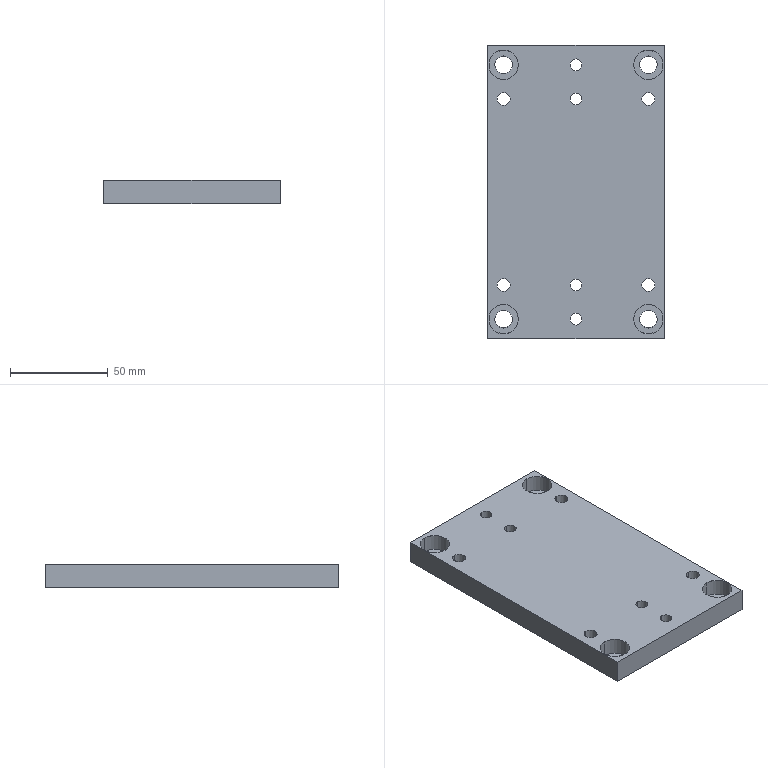Component | SolidWorks | X-AxisSliderShimPlate-1 | 1 solid | 102 faces | box 90 x 150 x 12 mm | volume 150499 mm3 | cone 48 | cylinder 40 | plane 14 | commonest cylinder face diameters 15 x8 9 x8 6 x8 11 x8 6.6 x8
build123d program:
from build123d import *

# Parameters (mm, degrees)
SKETCH1_W                                      = 150
SKETCH1_H                                      = 90
BOSS_EXTRUDE1_DEPTH                            = 12
SKETCH2_R                                      = 3
CUT_EXTRUDE1_DEPTH                             = 89.284
M6_HEX_SOCKET_HEAD_CAP_SCREW_CBORE1_AT_2_COUNT = 2
M6_HEX_SOCKET_HEAD_CAP_SCREW_CBORE1_AT_2_PITCH = 74
M6_HEX_SOCKET_HEAD_CAP_SCREW_CBORE1_AT_3_COUNT = 2
M6_HEX_SOCKET_HEAD_CAP_SCREW_CBORE1_AT_3_PITCH = 120.42
M6_HEX_SOCKET_HEAD_CAP_SCREW_CBORE1_AT_4_COUNT = 2
M6_HEX_SOCKET_HEAD_CAP_SCREW_CBORE1_AT_4_PITCH = 95
SKETCH5_R                                      = 3
CUT_EXTRUDE2_DEPTH                             = 89.284
M8_HEX_SOCKET_HEAD_CAP_SCREW_CBORE1_AT_2_COUNT = 2
M8_HEX_SOCKET_HEAD_CAP_SCREW_CBORE1_AT_2_PITCH = 130
M8_HEX_SOCKET_HEAD_CAP_SCREW_CBORE1_AT_3_COUNT = 2
M8_HEX_SOCKET_HEAD_CAP_SCREW_CBORE1_AT_3_PITCH = 149.586
M8_HEX_SOCKET_HEAD_CAP_SCREW_CBORE1_AT_4_COUNT = 2
M8_HEX_SOCKET_HEAD_CAP_SCREW_CBORE1_AT_4_PITCH = 74


with BuildPart() as part:
    # Sketch1 → Boss-Extrude1 (new body)
    with BuildSketch(Plane.XY):
        Rectangle(SKETCH1_W, SKETCH1_H)
    extrude(amount=BOSS_EXTRUDE1_DEPTH)

    # Sketch2 → Cut-Extrude1 (cut, through all)
    with BuildSketch(Plane.XY.offset(12)):
        with Locations((-47.5, 0)):
            Circle(SKETCH2_R)
        with Locations((47.5, 0)):
            Circle(SKETCH2_R)
    extrude(amount=-CUT_EXTRUDE1_DEPTH, mode=Mode.SUBTRACT)

    # Sketch3 → M6 Hex Socket Head Cap Screw CBORE1 (revolve, cut)
    with BuildSketch(Plane(origin=(-47.5, 37, 12), x_dir=(0, -1, 0), z_dir=(1, 0, 0))):
        Polygon((0, 0), (0, 12), (3.325, 12), (3.3, 11.975), (3.3, 6.425), (3.325, 6.4), (5.5, 6.4), (5.5, 0.025), (5.525, 0), align=None)
    m6_hex_socket_head_cap_screw_cbore1 = revolve(axis=Axis((-47.5, 37, 18.35), (0, 0, -1)), mode=Mode.SUBTRACT)

    # M6 Hex Socket Head Cap Screw CBORE1 at 2: M6 Hex Socket Head Cap Screw CBORE1 ×2
    with Locations(*[(0, -i * M6_HEX_SOCKET_HEAD_CAP_SCREW_CBORE1_AT_2_PITCH, 0) for i in range(1, M6_HEX_SOCKET_HEAD_CAP_SCREW_CBORE1_AT_2_COUNT)]):
        add(m6_hex_socket_head_cap_screw_cbore1, mode=Mode.SUBTRACT)

    # M6 Hex Socket Head Cap Screw CBORE1 at 3: M6 Hex Socket Head Cap Screw CBORE1 ×2
    with Locations(*[Vector(0.7889, -0.6145, 0) * (i * M6_HEX_SOCKET_HEAD_CAP_SCREW_CBORE1_AT_3_PITCH) for i in range(1, M6_HEX_SOCKET_HEAD_CAP_SCREW_CBORE1_AT_3_COUNT)]):
        add(m6_hex_socket_head_cap_screw_cbore1, mode=Mode.SUBTRACT)

    # M6 Hex Socket Head Cap Screw CBORE1 at 4: M6 Hex Socket Head Cap Screw CBORE1 ×2
    with Locations(*[(i * M6_HEX_SOCKET_HEAD_CAP_SCREW_CBORE1_AT_4_PITCH, 0, 0) for i in range(1, M6_HEX_SOCKET_HEAD_CAP_SCREW_CBORE1_AT_4_COUNT)]):
        add(m6_hex_socket_head_cap_screw_cbore1, mode=Mode.SUBTRACT)

    # Sketch5 → Cut-Extrude2 (cut, through all)
    with BuildSketch(Plane(origin=(0, 0, 0), x_dir=(-1, 0, 0), z_dir=(0, 0, -1))):
        with Locations((-65, 0)):
            Circle(SKETCH5_R)
        with Locations((65, 0)):
            Circle(SKETCH5_R)
    extrude(amount=-CUT_EXTRUDE2_DEPTH, mode=Mode.SUBTRACT)

    # Sketch6 → M8 Hex Socket Head Cap Screw CBORE1 (revolve, cut)
    with BuildSketch(Plane(origin=(65, 37, 0), x_dir=(0, 1, 0), z_dir=(1, 0, 0))):
        Polygon((0, 0), (0, 12), (4.525, 12), (4.5, 11.975), (4.5, 8.625), (4.525, 8.6), (7.5, 8.6), (7.5, 0.025), (7.525, 0), align=None)
    m8_hex_socket_head_cap_screw_cbore1 = revolve(axis=Axis((65, 37, -6.35), (0, 0, 1)), mode=Mode.SUBTRACT)

    # M8 Hex Socket Head Cap Screw CBORE1 at 2: M8 Hex Socket Head Cap Screw CBORE1 ×2
    with Locations(*[(-i * M8_HEX_SOCKET_HEAD_CAP_SCREW_CBORE1_AT_2_PITCH, 0, 0) for i in range(1, M8_HEX_SOCKET_HEAD_CAP_SCREW_CBORE1_AT_2_COUNT)]):
        add(m8_hex_socket_head_cap_screw_cbore1, mode=Mode.SUBTRACT)

    # M8 Hex Socket Head Cap Screw CBORE1 at 3: M8 Hex Socket Head Cap Screw CBORE1 ×2
    with Locations(*[Vector(-0.8691, -0.4947, 0) * (i * M8_HEX_SOCKET_HEAD_CAP_SCREW_CBORE1_AT_3_PITCH) for i in range(1, M8_HEX_SOCKET_HEAD_CAP_SCREW_CBORE1_AT_3_COUNT)]):
        add(m8_hex_socket_head_cap_screw_cbore1, mode=Mode.SUBTRACT)

    # M8 Hex Socket Head Cap Screw CBORE1 at 4: M8 Hex Socket Head Cap Screw CBORE1 ×2
    with Locations(*[(0, -i * M8_HEX_SOCKET_HEAD_CAP_SCREW_CBORE1_AT_4_PITCH, 0) for i in range(1, M8_HEX_SOCKET_HEAD_CAP_SCREW_CBORE1_AT_4_COUNT)]):
        add(m8_hex_socket_head_cap_screw_cbore1, mode=Mode.SUBTRACT)


solid = part.part

# Placed as in the assembly
solid = solid.moved(Location((19.229, 0, -0.5), (180, 0, -90)))